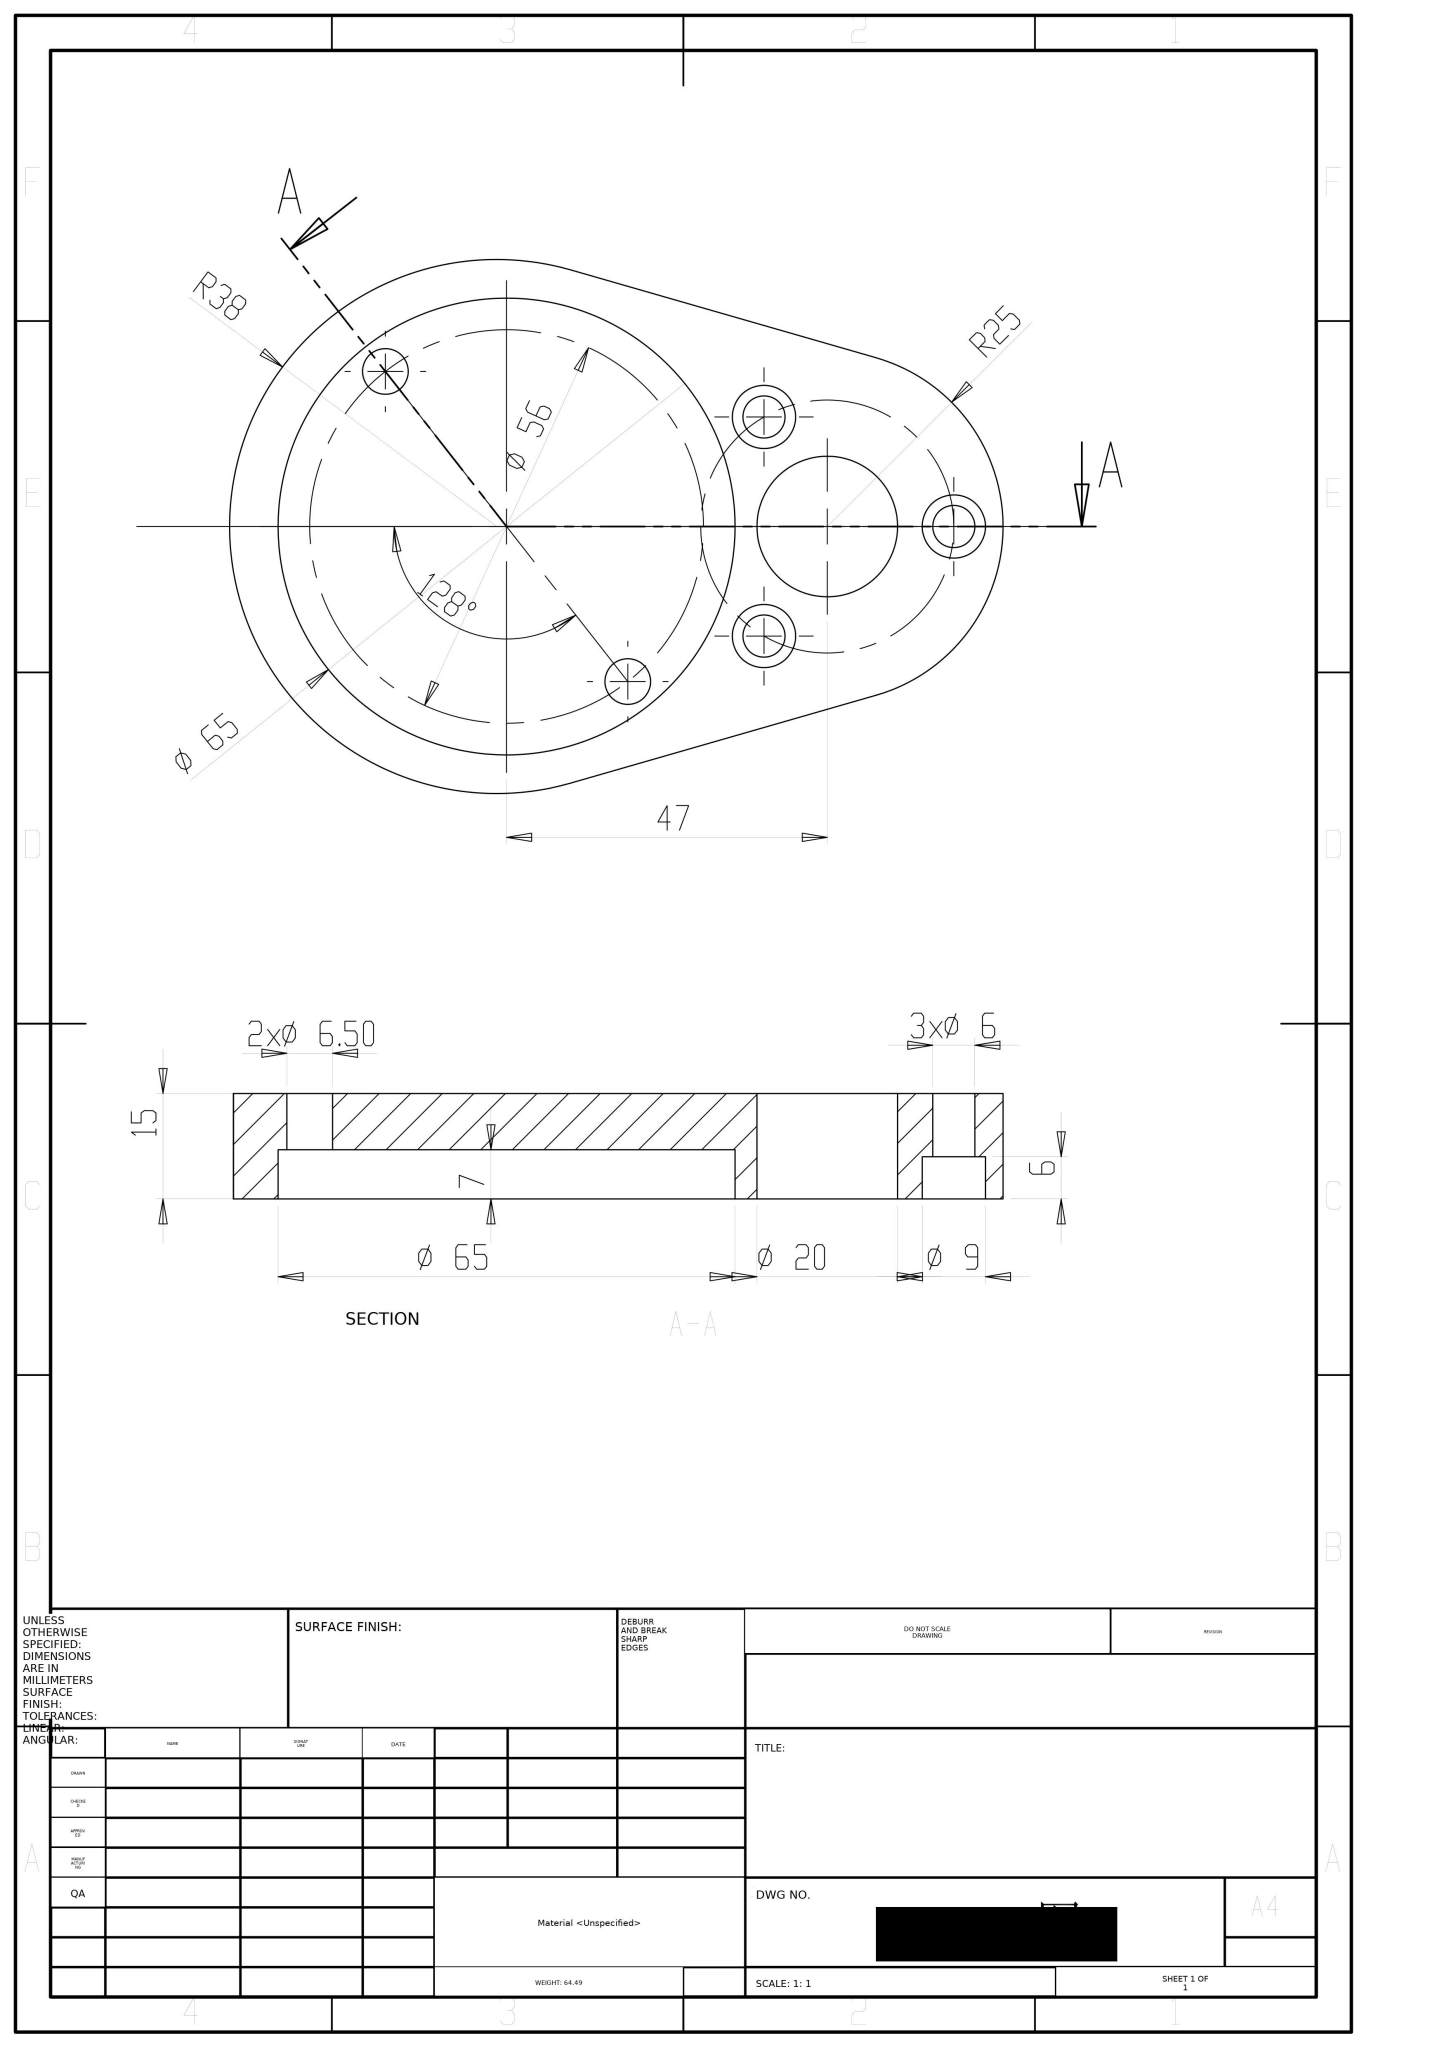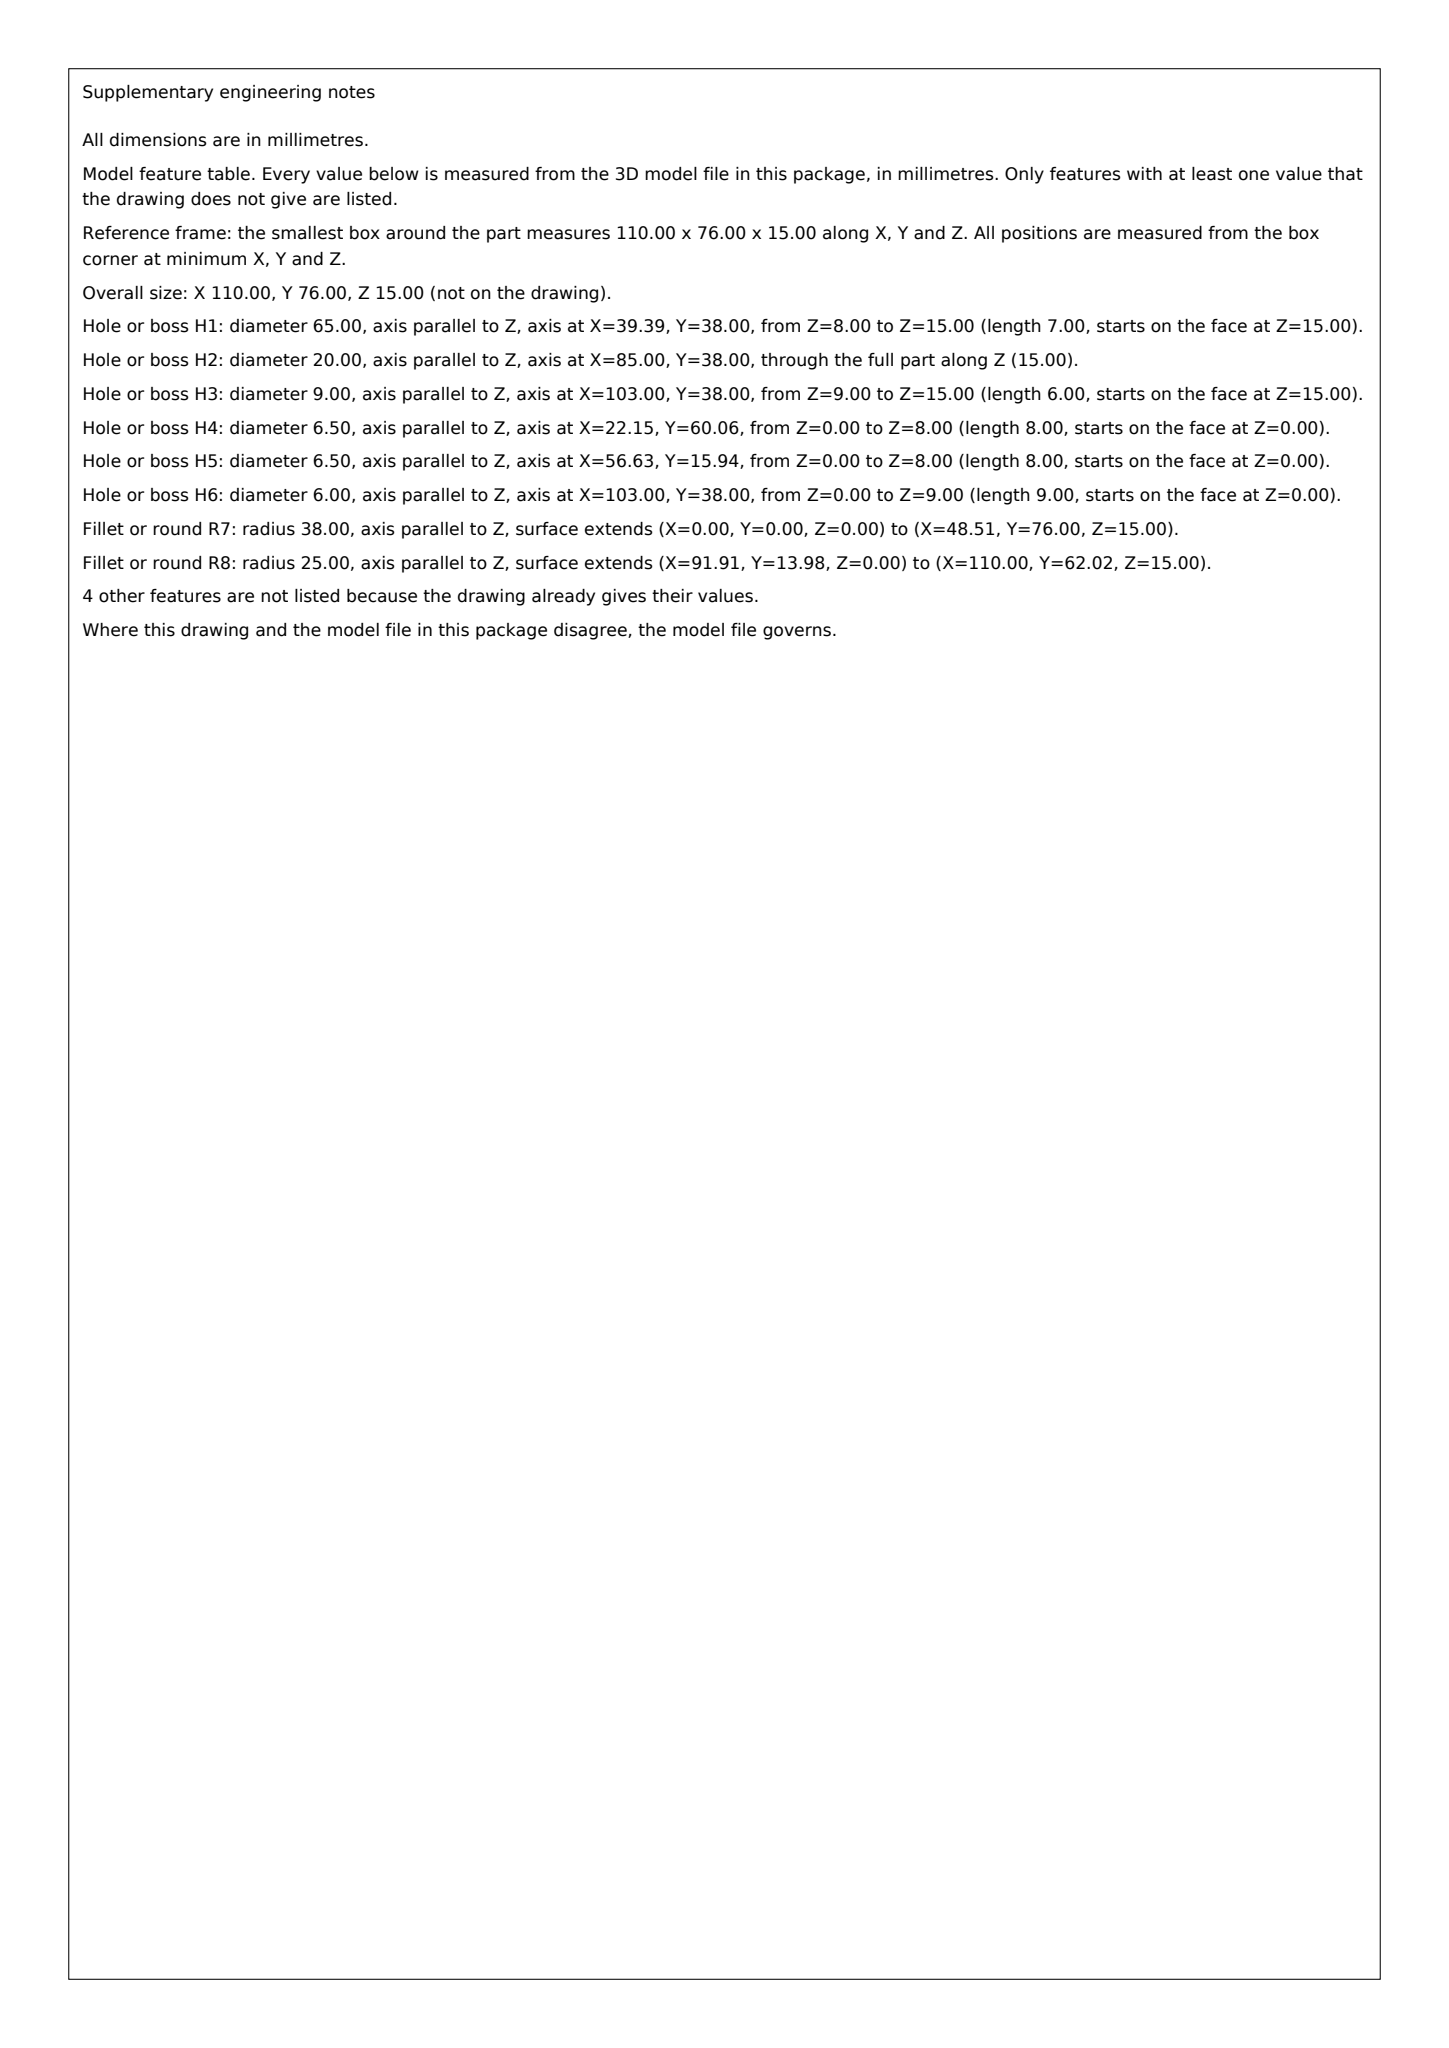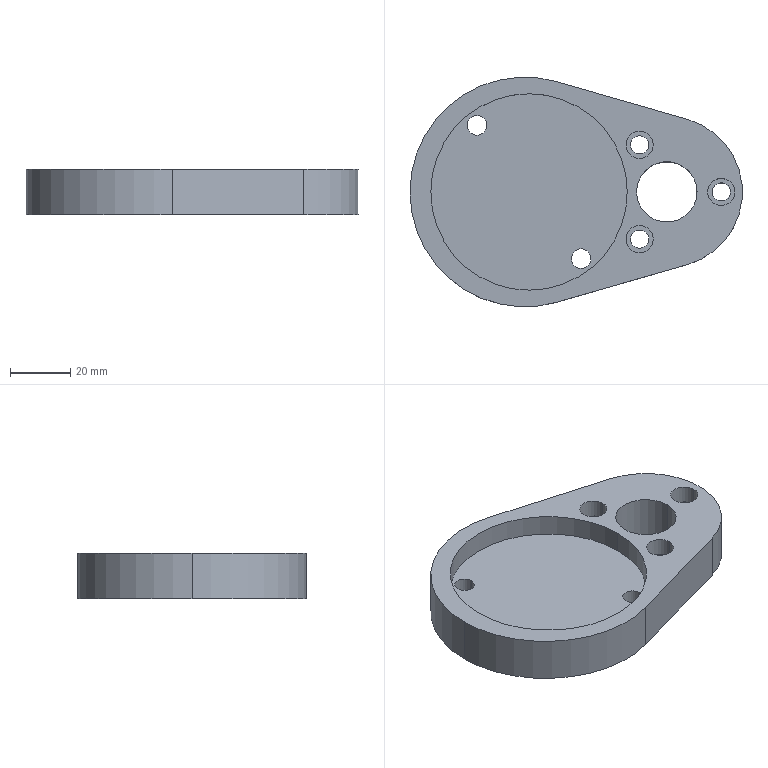Part | SolidWorks | mm | 1 solid | 31 faces | box 110 x 76 x 15 mm | volume 64495 mm3 | cylinder 23 | plane 8 | commonest cylinder face diameters 6 x6 9 x6 6.5 x4 20 x2 65 x2 76 x2 50 x1
build123d program:
from build123d import *

# Parameters (mm, degrees)
BOSS_EXTRUDE1_DEPTH = 15
SKETCH2_R           = 32.5
CUT_EXTRUDE1_DEPTH  = 7
SKETCH4_R           = 3.25
CUT_EXTRUDE2_DEPTH  = 81.581
SKETCH5_R           = 10
CUT_EXTRUDE3_DEPTH  = 82.574
SKETCH6_R           = 4.5
CUT_EXTRUDE4_DEPTH  = 6
SKETCH7_R           = 3
CUT_EXTRUDE5_DEPTH  = 81.687


with BuildPart() as part:
    # Sketch1 → Boss-Extrude1 (new body)
    with BuildSketch(Plane.XY):
        with BuildLine():
            Line((9.118, 36.517), (52.522, 24.025))
            ThreePointArc((52.522, 24.025), (70.607, 0), (52.522, -24.025))
            Line((52.522, -24.025), (9.118, -36.517))
            ThreePointArc((9.118, -36.517), (-39.393, 0), (9.118, 36.517))
        make_face()
    extrude(amount=BOSS_EXTRUDE1_DEPTH)

    # Sketch2 → Cut-Extrude1 (cut)
    with BuildSketch(Plane.XY.offset(15)):
        Circle(SKETCH2_R)
    extrude(amount=-CUT_EXTRUDE1_DEPTH, mode=Mode.SUBTRACT)

    # Sketch4 → Cut-Extrude2 (cut, through all)
    with BuildSketch(Plane.XY.offset(8)):
        with Locations((17.239, -22.064)):
            Circle(SKETCH4_R)
        with Locations((-17.239, 22.064)):
            Circle(SKETCH4_R)
    extrude(amount=-CUT_EXTRUDE2_DEPTH, mode=Mode.SUBTRACT)

    # Sketch5 → Cut-Extrude3 (cut, through all)
    with BuildSketch(Plane.XY.offset(15)):
        with Locations((45.607, 0)):
            Circle(SKETCH5_R)
    extrude(amount=-CUT_EXTRUDE3_DEPTH, mode=Mode.SUBTRACT)

    # Sketch6 → Cut-Extrude4 (cut)
    with BuildSketch(Plane.XY.offset(15)):
        with Locations((63.607, 0)):
            Circle(SKETCH6_R)
        with Locations((36.607, -15.588)):
            Circle(SKETCH6_R)
        with Locations((36.607, 15.588)):
            Circle(SKETCH6_R)
    extrude(amount=-CUT_EXTRUDE4_DEPTH, mode=Mode.SUBTRACT)

    # Sketch7 → Cut-Extrude5 (cut, through all)
    with BuildSketch(Plane.XY.offset(9)):
        with Locations((63.607, 0)):
            Circle(SKETCH7_R)
        with Locations((36.607, -15.588)):
            Circle(SKETCH7_R)
        with Locations((36.607, 15.588)):
            Circle(SKETCH7_R)
    extrude(amount=-CUT_EXTRUDE5_DEPTH, mode=Mode.SUBTRACT)


solid = part.part